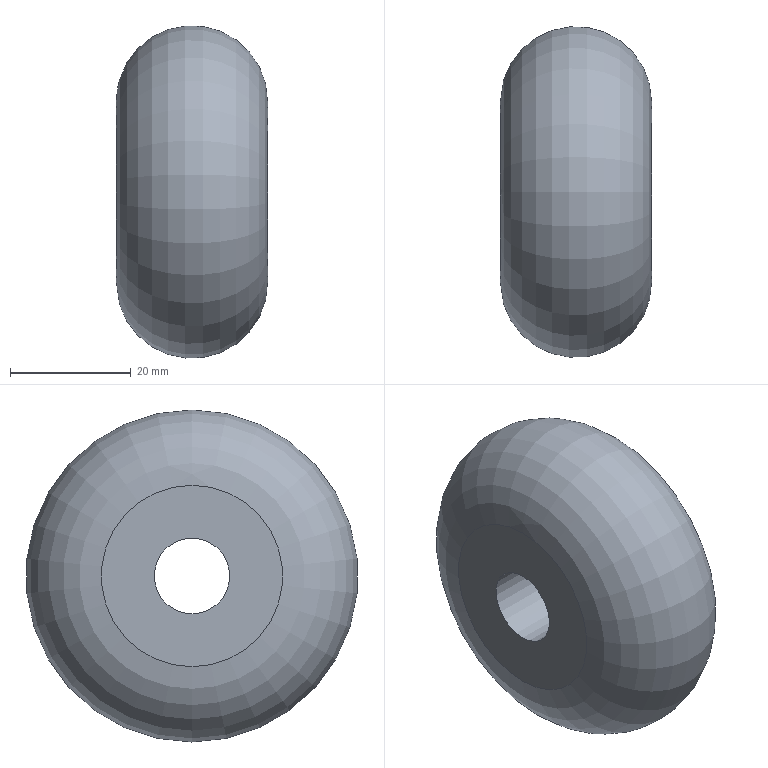Component | NX | HANDLE | 1 solid | 4 faces | box 25 x 55 x 55 mm | volume 45917 mm3 | plane 2 | torus 1 | cylinder 1 | commonest cylinder face diameters 12.5 x1
STEP:
#1=CARTESIAN_POINT('',(0.,0.,0.));
#2=DIRECTION('',(0.,0.,1.));
#3=DIRECTION('',(1.,0.,0.));
#4=AXIS2_PLACEMENT_3D('',#1,#2,#3);
#5=CARTESIAN_POINT('',(-160.,-0.,207.75));
#6=VERTEX_POINT('',#5);
#7=CARTESIAN_POINT('',(-160.,-0.,201.5));
#8=DIRECTION('',(-1.,0.,0.));
#9=DIRECTION('',(0.,0.,1.));
#10=AXIS2_PLACEMENT_3D('',#7,#8,#9);
#11=CIRCLE('',#10,6.25);
#12=CARTESIAN_POINT('',(-160.,-0.,216.5));
#13=DIRECTION('',(1.,0.,0.));
#14=DIRECTION('',(0.,0.,-1.));
#15=AXIS2_PLACEMENT_3D('',#12,#13,#14);
#16=PLANE('',#15);
#17=CARTESIAN_POINT('',(8.75,0.));
#18=CARTESIAN_POINT('',(8.75,10.825));
#19=CARTESIAN_POINT('',(18.125,5.413));
#20=CARTESIAN_POINT('',(27.5,0.));
#21=CARTESIAN_POINT('',(18.125,-5.413));
#22=CARTESIAN_POINT('',(8.75,-10.825));
#23=CARTESIAN_POINT('',(8.75,0.));
#24=(BOUNDED_CURVE()B_SPLINE_CURVE(2,(#17,#18,#19,#20,#21,#22,#23),.UNSPECIFIED.,.T.,.F.)B_SPLINE_CURVE_WITH_KNOTS((1,2,2,2,2,1),(-2.094,0.,2.094,4.189,6.283,8.378),.UNSPECIFIED.)CURVE()GEOMETRIC_REPRESENTATION_ITEM()RATIONAL_B_SPLINE_CURVE((1.,0.5,1.,0.5,1.,0.5,1.))REPRESENTATION_ITEM(''));
#25=(GEOMETRIC_REPRESENTATION_CONTEXT(2)PARAMETRIC_REPRESENTATION_CONTEXT()REPRESENTATION_CONTEXT('',''));
#26=DEFINITIONAL_REPRESENTATION('',(#24),#25);
#27=PCURVE('',#16,#26);
#28=CARTESIAN_POINT('',(-160.,-0.,201.5));
#29=DIRECTION('',(-1.,0.,0.));
#30=DIRECTION('',(0.,0.,1.));
#31=AXIS2_PLACEMENT_3D('',#28,#29,#30);
#32=CYLINDRICAL_SURFACE('',#31,6.25);
#33=CARTESIAN_POINT('',(0.,0.));
#34=DIRECTION('',(1.,0.));
#35=VECTOR('',#34,1.);
#36=LINE('',#33,#35);
#37=(GEOMETRIC_REPRESENTATION_CONTEXT(2)PARAMETRIC_REPRESENTATION_CONTEXT()REPRESENTATION_CONTEXT('',''));
#38=DEFINITIONAL_REPRESENTATION('',(#36),#37);
#39=PCURVE('',#32,#38);
#40=SURFACE_CURVE('',#11,(#27,#39),.PCURVE_S1.);
#41=EDGE_CURVE('',#6,#6,#40,.T.);
#42=ORIENTED_EDGE('',*,*,#41,.T.);
#43=EDGE_LOOP('',(#42));
#44=FACE_BOUND('',#43,.T.);
#45=CARTESIAN_POINT('',(-160.,-0.,216.5));
#46=VERTEX_POINT('',#45);
#47=CARTESIAN_POINT('',(-160.,-0.,201.5));
#48=DIRECTION('',(-1.,0.,0.));
#49=DIRECTION('',(0.,0.,1.));
#50=AXIS2_PLACEMENT_3D('',#47,#48,#49);
#51=CIRCLE('',#50,15.);
#52=CARTESIAN_POINT('',(0.,0.));
#53=CARTESIAN_POINT('',(0.,25.981));
#54=CARTESIAN_POINT('',(22.5,12.99));
#55=CARTESIAN_POINT('',(45.,0.));
#56=CARTESIAN_POINT('',(22.5,-12.99));
#57=CARTESIAN_POINT('',(0.,-25.981));
#58=CARTESIAN_POINT('',(0.,0.));
#59=(BOUNDED_CURVE()B_SPLINE_CURVE(2,(#52,#53,#54,#55,#56,#57,#58),.UNSPECIFIED.,.T.,.F.)B_SPLINE_CURVE_WITH_KNOTS((1,2,2,2,2,1),(-2.094,0.,2.094,4.189,6.283,8.378),.UNSPECIFIED.)CURVE()GEOMETRIC_REPRESENTATION_ITEM()RATIONAL_B_SPLINE_CURVE((1.,0.5,1.,0.5,1.,0.5,1.))REPRESENTATION_ITEM(''));
#60=(GEOMETRIC_REPRESENTATION_CONTEXT(2)PARAMETRIC_REPRESENTATION_CONTEXT()REPRESENTATION_CONTEXT('',''));
#61=DEFINITIONAL_REPRESENTATION('',(#59),#60);
#62=PCURVE('',#16,#61);
#63=CARTESIAN_POINT('',(-172.5,-0.,201.5));
#64=DIRECTION('',(-1.,0.,0.));
#65=DIRECTION('',(0.,0.,1.));
#66=AXIS2_PLACEMENT_3D('',#63,#64,#65);
#67=TOROIDAL_SURFACE('',#66,15.,12.5);
#68=CARTESIAN_POINT('',(0.,4.712));
#69=DIRECTION('',(1.,0.));
#70=VECTOR('',#69,1.);
#71=LINE('',#68,#70);
#72=(GEOMETRIC_REPRESENTATION_CONTEXT(2)PARAMETRIC_REPRESENTATION_CONTEXT()REPRESENTATION_CONTEXT('',''));
#73=DEFINITIONAL_REPRESENTATION('',(#71),#72);
#74=PCURVE('',#67,#73);
#75=SURFACE_CURVE('',#51,(#62,#74),.PCURVE_S1.);
#76=EDGE_CURVE('',#46,#46,#75,.T.);
#77=ORIENTED_EDGE('',*,*,#76,.F.);
#78=EDGE_LOOP('',(#77));
#79=FACE_BOUND('',#78,.T.);
#80=ADVANCED_FACE('',(#44,#79),#16,.T.);
#81=ORIENTED_EDGE('',*,*,#76,.T.);
#82=CARTESIAN_POINT('',(-185.,-0.,216.5));
#83=VERTEX_POINT('',#82);
#84=CARTESIAN_POINT('',(-160.,-0.,216.5));
#85=CARTESIAN_POINT('',(-160.,-0.,220.863));
#86=CARTESIAN_POINT('',(-161.713,-0.,225.227));
#87=CARTESIAN_POINT('',(-165.14,-0.,228.821));
#88=CARTESIAN_POINT('',(-169.878,-0.,230.878));
#89=CARTESIAN_POINT('',(-175.122,-0.,230.878));
#90=CARTESIAN_POINT('',(-179.86,-0.,228.821));
#91=CARTESIAN_POINT('',(-183.287,-0.,225.227));
#92=CARTESIAN_POINT('',(-185.,-0.,220.863));
#93=CARTESIAN_POINT('',(-185.,-0.,216.5));
#94=B_SPLINE_CURVE_WITH_KNOTS('',9,(#84,#85,#86,#87,#88,#89,#90,#91,#92,#93),.UNSPECIFIED.,.F.,.F.,(10,10),(4.712,7.854),.PIECEWISE_BEZIER_KNOTS.);
#95=CARTESIAN_POINT('',(6.283,0.));
#96=DIRECTION('',(0.,1.));
#97=VECTOR('',#96,1.);
#98=LINE('',#95,#97);
#99=(GEOMETRIC_REPRESENTATION_CONTEXT(2)PARAMETRIC_REPRESENTATION_CONTEXT()REPRESENTATION_CONTEXT('',''));
#100=DEFINITIONAL_REPRESENTATION('',(#98),#99);
#101=PCURVE('',#67,#100);
#102=CARTESIAN_POINT('',(0.,0.));
#103=DIRECTION('',(0.,1.));
#104=VECTOR('',#103,1.);
#105=LINE('',#102,#104);
#106=(GEOMETRIC_REPRESENTATION_CONTEXT(2)PARAMETRIC_REPRESENTATION_CONTEXT()REPRESENTATION_CONTEXT('',''));
#107=DEFINITIONAL_REPRESENTATION('',(#105),#106);
#108=PCURVE('',#67,#107);
#109=SEAM_CURVE('',#94,(#101,#108),.PCURVE_S1.);
#110=EDGE_CURVE('',#46,#83,#109,.T.);
#111=ORIENTED_EDGE('',*,*,#110,.T.);
#112=CARTESIAN_POINT('',(-185.,-0.,201.5));
#113=DIRECTION('',(-1.,0.,0.));
#114=DIRECTION('',(0.,0.,1.));
#115=AXIS2_PLACEMENT_3D('',#112,#113,#114);
#116=CIRCLE('',#115,15.);
#117=CARTESIAN_POINT('',(0.,7.854));
#118=DIRECTION('',(1.,0.));
#119=VECTOR('',#118,1.);
#120=LINE('',#117,#119);
#121=(GEOMETRIC_REPRESENTATION_CONTEXT(2)PARAMETRIC_REPRESENTATION_CONTEXT()REPRESENTATION_CONTEXT('',''));
#122=DEFINITIONAL_REPRESENTATION('',(#120),#121);
#123=PCURVE('',#67,#122);
#124=CARTESIAN_POINT('',(-185.,-0.,201.5));
#125=DIRECTION('',(-1.,0.,0.));
#126=DIRECTION('',(0.,0.,1.));
#127=AXIS2_PLACEMENT_3D('',#124,#125,#126);
#128=PLANE('',#127);
#129=CARTESIAN_POINT('',(0.,0.));
#130=DIRECTION('',(1.,0.));
#131=AXIS2_PLACEMENT_2D('',#129,#130);
#132=CIRCLE('',#131,15.);
#133=(GEOMETRIC_REPRESENTATION_CONTEXT(2)PARAMETRIC_REPRESENTATION_CONTEXT()REPRESENTATION_CONTEXT('',''));
#134=DEFINITIONAL_REPRESENTATION('',(#132),#133);
#135=PCURVE('',#128,#134);
#136=SURFACE_CURVE('',#116,(#123,#135),.PCURVE_S1.);
#137=EDGE_CURVE('',#83,#83,#136,.T.);
#138=ORIENTED_EDGE('',*,*,#137,.F.);
#139=ORIENTED_EDGE('',*,*,#110,.F.);
#140=EDGE_LOOP('',(#81,#111,#138,#139));
#141=FACE_BOUND('',#140,.T.);
#142=ADVANCED_FACE('',(#141),#67,.T.);
#143=CARTESIAN_POINT('',(-185.,-0.,207.75));
#144=VERTEX_POINT('',#143);
#145=CARTESIAN_POINT('',(-185.,-0.,201.5));
#146=DIRECTION('',(-1.,0.,0.));
#147=DIRECTION('',(0.,0.,1.));
#148=AXIS2_PLACEMENT_3D('',#145,#146,#147);
#149=CIRCLE('',#148,6.25);
#150=CARTESIAN_POINT('',(0.,0.));
#151=DIRECTION('',(1.,0.));
#152=AXIS2_PLACEMENT_2D('',#150,#151);
#153=CIRCLE('',#152,6.25);
#154=(GEOMETRIC_REPRESENTATION_CONTEXT(2)PARAMETRIC_REPRESENTATION_CONTEXT()REPRESENTATION_CONTEXT('',''));
#155=DEFINITIONAL_REPRESENTATION('',(#153),#154);
#156=PCURVE('',#128,#155);
#157=CARTESIAN_POINT('',(0.,25.));
#158=DIRECTION('',(1.,0.));
#159=VECTOR('',#158,1.);
#160=LINE('',#157,#159);
#161=(GEOMETRIC_REPRESENTATION_CONTEXT(2)PARAMETRIC_REPRESENTATION_CONTEXT()REPRESENTATION_CONTEXT('',''));
#162=DEFINITIONAL_REPRESENTATION('',(#160),#161);
#163=PCURVE('',#32,#162);
#164=SURFACE_CURVE('',#149,(#156,#163),.PCURVE_S1.);
#165=EDGE_CURVE('',#144,#144,#164,.T.);
#166=ORIENTED_EDGE('',*,*,#165,.F.);
#167=EDGE_LOOP('',(#166));
#168=FACE_BOUND('',#167,.T.);
#169=ORIENTED_EDGE('',*,*,#137,.T.);
#170=EDGE_LOOP('',(#169));
#171=FACE_BOUND('',#170,.T.);
#172=ADVANCED_FACE('',(#168,#171),#128,.T.);
#173=ORIENTED_EDGE('',*,*,#165,.F.);
#174=CARTESIAN_POINT('',(-160.,-0.,207.75));
#175=CARTESIAN_POINT('',(-185.,-0.,207.75));
#176=B_SPLINE_CURVE_WITH_KNOTS('',1,(#174,#175),.UNSPECIFIED.,.F.,.F.,(2,2),(0.,25.),.PIECEWISE_BEZIER_KNOTS.);
#177=CARTESIAN_POINT('',(0.,0.));
#178=DIRECTION('',(0.,1.));
#179=VECTOR('',#178,1.);
#180=LINE('',#177,#179);
#181=(GEOMETRIC_REPRESENTATION_CONTEXT(2)PARAMETRIC_REPRESENTATION_CONTEXT()REPRESENTATION_CONTEXT('',''));
#182=DEFINITIONAL_REPRESENTATION('',(#180),#181);
#183=PCURVE('',#32,#182);
#184=CARTESIAN_POINT('',(6.283,0.));
#185=DIRECTION('',(0.,1.));
#186=VECTOR('',#185,1.);
#187=LINE('',#184,#186);
#188=(GEOMETRIC_REPRESENTATION_CONTEXT(2)PARAMETRIC_REPRESENTATION_CONTEXT()REPRESENTATION_CONTEXT('',''));
#189=DEFINITIONAL_REPRESENTATION('',(#187),#188);
#190=PCURVE('',#32,#189);
#191=SEAM_CURVE('',#176,(#183,#190),.PCURVE_S1.);
#192=EDGE_CURVE('',#6,#144,#191,.T.);
#193=ORIENTED_EDGE('',*,*,#192,.F.);
#194=ORIENTED_EDGE('',*,*,#41,.T.);
#195=ORIENTED_EDGE('',*,*,#192,.T.);
#196=EDGE_LOOP('',(#173,#193,#194,#195));
#197=FACE_BOUND('',#196,.F.);
#198=ADVANCED_FACE('',(#197),#32,.F.);
#199=CLOSED_SHELL('',(#80,#142,#172,#198));
#200=MANIFOLD_SOLID_BREP('',#199);
#201=(LENGTH_UNIT()NAMED_UNIT(*)SI_UNIT(.MILLI.,.METRE.));
#202=UNCERTAINTY_MEASURE_WITH_UNIT(LENGTH_MEASURE(0.00001),#201,'','');
#203=(NAMED_UNIT(*)PLANE_ANGLE_UNIT()SI_UNIT($,.RADIAN.));
#204=(NAMED_UNIT(*)SI_UNIT($,.STERADIAN.)SOLID_ANGLE_UNIT());
#205=(GEOMETRIC_REPRESENTATION_CONTEXT(3)GLOBAL_UNCERTAINTY_ASSIGNED_CONTEXT((#202))GLOBAL_UNIT_ASSIGNED_CONTEXT((#201,#203,#204))REPRESENTATION_CONTEXT('',''));
#206=ADVANCED_BREP_SHAPE_REPRESENTATION('',(#4,#200),#205);